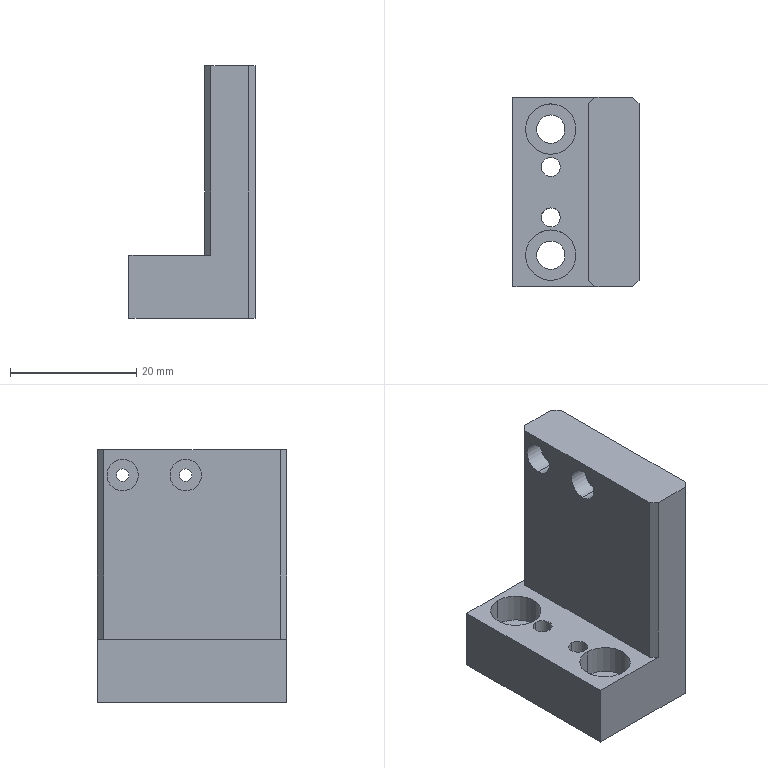Component | SolidWorks | JQ-2-0-007-3 | 1 solid | 36 faces | box 20 x 30 x 40 mm | volume 12205 mm3 | cylinder 20 | plane 16 | commonest cylinder face diameters 3 x4 2 x4 5 x4 8 x4 4.5 x4
STEP:
#1=COLOUR_RGB('',0.7922,0.8196,0.9333);
#2=FILL_AREA_STYLE_COLOUR('',#1);
#3=FILL_AREA_STYLE('',(#2));
#4=SURFACE_STYLE_FILL_AREA(#3);
#5=SURFACE_SIDE_STYLE('',(#4));
#6=SURFACE_STYLE_USAGE(.BOTH.,#5);
#7=PRESENTATION_STYLE_ASSIGNMENT((#6));
#8=CARTESIAN_POINT('',(-7.994,0.9385,4.611));
#9=VERTEX_POINT('',#8);
#10=CARTESIAN_POINT('',(-7.994,1.057,4.611));
#11=VERTEX_POINT('',#10);
#12=CARTESIAN_POINT('',(-7.994,0.9976,4.611));
#13=DIRECTION('',(0.,0.,1.));
#14=DIRECTION('',(0.,1.,0.));
#15=AXIS2_PLACEMENT_3D('',#12,#13,#14);
#16=CIRCLE('',#15,0.05906);
#17=EDGE_CURVE('',#9,#11,#16,.T.);
#18=ORIENTED_EDGE('',*,*,#17,.F.);
#19=CARTESIAN_POINT('',(-7.994,0.9385,5.005));
#20=VERTEX_POINT('',#19);
#21=CARTESIAN_POINT('',(-7.994,0.9385,4.611));
#22=DIRECTION('',(0.,0.,1.));
#23=VECTOR('',#22,39.37);
#24=LINE('',#21,#23);
#25=EDGE_CURVE('',#9,#20,#24,.T.);
#26=ORIENTED_EDGE('',*,*,#25,.T.);
#27=CARTESIAN_POINT('',(-7.994,1.057,5.005));
#28=VERTEX_POINT('',#27);
#29=CARTESIAN_POINT('',(-7.994,0.9976,5.005));
#30=DIRECTION('',(0.,0.,1.));
#31=DIRECTION('',(0.,1.,0.));
#32=AXIS2_PLACEMENT_3D('',#29,#30,#31);
#33=CIRCLE('',#32,0.05906);
#34=EDGE_CURVE('',#20,#28,#33,.T.);
#35=ORIENTED_EDGE('',*,*,#34,.T.);
#36=CARTESIAN_POINT('',(-7.994,1.057,4.611));
#37=DIRECTION('',(0.,0.,1.));
#38=VECTOR('',#37,39.37);
#39=LINE('',#36,#38);
#40=EDGE_CURVE('',#11,#28,#39,.T.);
#41=ORIENTED_EDGE('',*,*,#40,.F.);
#42=EDGE_LOOP('',(#18,#26,#35,#41));
#43=FACE_OUTER_BOUND('',#42,.T.);
#44=CARTESIAN_POINT('',(-7.994,0.9976,4.611));
#45=DIRECTION('',(0.,0.,1.));
#46=DIRECTION('',(0.,1.,0.));
#47=AXIS2_PLACEMENT_3D('',#44,#45,#46);
#48=CYLINDRICAL_SURFACE('',#47,0.05906);
#49=ADVANCED_FACE('',(#43),#48,.F.);
#50=CARTESIAN_POINT('',(-7.994,1.254,4.611));
#51=VERTEX_POINT('',#50);
#52=CARTESIAN_POINT('',(-7.994,1.372,4.611));
#53=VERTEX_POINT('',#52);
#54=CARTESIAN_POINT('',(-7.994,1.313,4.611));
#55=DIRECTION('',(0.,0.,1.));
#56=DIRECTION('',(0.,1.,0.));
#57=AXIS2_PLACEMENT_3D('',#54,#55,#56);
#58=CIRCLE('',#57,0.05906);
#59=EDGE_CURVE('',#51,#53,#58,.T.);
#60=ORIENTED_EDGE('',*,*,#59,.F.);
#61=CARTESIAN_POINT('',(-7.994,1.254,5.005));
#62=VERTEX_POINT('',#61);
#63=CARTESIAN_POINT('',(-7.994,1.254,4.611));
#64=DIRECTION('',(0.,0.,1.));
#65=VECTOR('',#64,39.37);
#66=LINE('',#63,#65);
#67=EDGE_CURVE('',#51,#62,#66,.T.);
#68=ORIENTED_EDGE('',*,*,#67,.T.);
#69=CARTESIAN_POINT('',(-7.994,1.372,5.005));
#70=VERTEX_POINT('',#69);
#71=CARTESIAN_POINT('',(-7.994,1.313,5.005));
#72=DIRECTION('',(0.,0.,1.));
#73=DIRECTION('',(0.,1.,0.));
#74=AXIS2_PLACEMENT_3D('',#71,#72,#73);
#75=CIRCLE('',#74,0.05906);
#76=EDGE_CURVE('',#62,#70,#75,.T.);
#77=ORIENTED_EDGE('',*,*,#76,.T.);
#78=CARTESIAN_POINT('',(-7.994,1.372,4.611));
#79=DIRECTION('',(0.,0.,1.));
#80=VECTOR('',#79,39.37);
#81=LINE('',#78,#80);
#82=EDGE_CURVE('',#53,#70,#81,.T.);
#83=ORIENTED_EDGE('',*,*,#82,.F.);
#84=EDGE_LOOP('',(#60,#68,#77,#83));
#85=FACE_OUTER_BOUND('',#84,.T.);
#86=CARTESIAN_POINT('',(-7.994,1.313,4.611));
#87=DIRECTION('',(0.,0.,1.));
#88=DIRECTION('',(0.,1.,0.));
#89=AXIS2_PLACEMENT_3D('',#86,#87,#88);
#90=CYLINDRICAL_SURFACE('',#89,0.05906);
#91=ADVANCED_FACE('',(#85),#90,.F.);
#92=CARTESIAN_POINT('',(-7.443,1.194,5.989));
#93=VERTEX_POINT('',#92);
#94=CARTESIAN_POINT('',(-7.443,1.194,6.068));
#95=VERTEX_POINT('',#94);
#96=CARTESIAN_POINT('',(-7.443,1.194,6.029));
#97=DIRECTION('',(-1.,-0.,0.));
#98=DIRECTION('',(0.,0.,1.));
#99=AXIS2_PLACEMENT_3D('',#96,#97,#98);
#100=CIRCLE('',#99,0.03937);
#101=EDGE_CURVE('',#93,#95,#100,.T.);
#102=ORIENTED_EDGE('',*,*,#101,.F.);
#103=CARTESIAN_POINT('',(-7.64,1.194,5.989));
#104=VERTEX_POINT('',#103);
#105=CARTESIAN_POINT('',(-7.443,1.194,5.989));
#106=DIRECTION('',(-1.,-0.,0.));
#107=VECTOR('',#106,39.37);
#108=LINE('',#105,#107);
#109=EDGE_CURVE('',#93,#104,#108,.T.);
#110=ORIENTED_EDGE('',*,*,#109,.T.);
#111=CARTESIAN_POINT('',(-7.64,1.194,6.068));
#112=VERTEX_POINT('',#111);
#113=CARTESIAN_POINT('',(-7.64,1.194,6.029));
#114=DIRECTION('',(-1.,-0.,0.));
#115=DIRECTION('',(0.,0.,1.));
#116=AXIS2_PLACEMENT_3D('',#113,#114,#115);
#117=CIRCLE('',#116,0.03937);
#118=EDGE_CURVE('',#104,#112,#117,.T.);
#119=ORIENTED_EDGE('',*,*,#118,.T.);
#120=CARTESIAN_POINT('',(-7.443,1.194,6.068));
#121=DIRECTION('',(-1.,-0.,0.));
#122=VECTOR('',#121,39.37);
#123=LINE('',#120,#122);
#124=EDGE_CURVE('',#95,#112,#123,.T.);
#125=ORIENTED_EDGE('',*,*,#124,.F.);
#126=EDGE_LOOP('',(#102,#110,#119,#125));
#127=FACE_OUTER_BOUND('',#126,.T.);
#128=CARTESIAN_POINT('',(-7.443,1.194,6.029));
#129=DIRECTION('',(-1.,-0.,0.));
#130=DIRECTION('',(0.,0.,1.));
#131=AXIS2_PLACEMENT_3D('',#128,#129,#130);
#132=CYLINDRICAL_SURFACE('',#131,0.03937);
#133=ADVANCED_FACE('',(#127),#132,.F.);
#134=CARTESIAN_POINT('',(-7.443,1.588,5.989));
#135=VERTEX_POINT('',#134);
#136=CARTESIAN_POINT('',(-7.443,1.588,6.068));
#137=VERTEX_POINT('',#136);
#138=CARTESIAN_POINT('',(-7.443,1.588,6.029));
#139=DIRECTION('',(-1.,-0.,0.));
#140=DIRECTION('',(0.,0.,1.));
#141=AXIS2_PLACEMENT_3D('',#138,#139,#140);
#142=CIRCLE('',#141,0.03937);
#143=EDGE_CURVE('',#135,#137,#142,.T.);
#144=ORIENTED_EDGE('',*,*,#143,.F.);
#145=CARTESIAN_POINT('',(-7.64,1.588,5.989));
#146=VERTEX_POINT('',#145);
#147=CARTESIAN_POINT('',(-7.443,1.588,5.989));
#148=DIRECTION('',(-1.,-0.,0.));
#149=VECTOR('',#148,39.37);
#150=LINE('',#147,#149);
#151=EDGE_CURVE('',#135,#146,#150,.T.);
#152=ORIENTED_EDGE('',*,*,#151,.T.);
#153=CARTESIAN_POINT('',(-7.64,1.588,6.068));
#154=VERTEX_POINT('',#153);
#155=CARTESIAN_POINT('',(-7.64,1.588,6.029));
#156=DIRECTION('',(-1.,-0.,0.));
#157=DIRECTION('',(0.,0.,1.));
#158=AXIS2_PLACEMENT_3D('',#155,#156,#157);
#159=CIRCLE('',#158,0.03937);
#160=EDGE_CURVE('',#146,#154,#159,.T.);
#161=ORIENTED_EDGE('',*,*,#160,.T.);
#162=CARTESIAN_POINT('',(-7.443,1.588,6.068));
#163=DIRECTION('',(-1.,-0.,0.));
#164=VECTOR('',#163,39.37);
#165=LINE('',#162,#164);
#166=EDGE_CURVE('',#137,#154,#165,.T.);
#167=ORIENTED_EDGE('',*,*,#166,.F.);
#168=EDGE_LOOP('',(#144,#152,#161,#167));
#169=FACE_OUTER_BOUND('',#168,.T.);
#170=CARTESIAN_POINT('',(-7.443,1.588,6.029));
#171=DIRECTION('',(-1.,-0.,0.));
#172=DIRECTION('',(0.,0.,1.));
#173=AXIS2_PLACEMENT_3D('',#170,#171,#172);
#174=CYLINDRICAL_SURFACE('',#173,0.03937);
#175=ADVANCED_FACE('',(#169),#174,.F.);
#176=CARTESIAN_POINT('',(-7.64,1.194,5.93));
#177=VERTEX_POINT('',#176);
#178=CARTESIAN_POINT('',(-7.64,1.194,6.127));
#179=VERTEX_POINT('',#178);
#180=CARTESIAN_POINT('',(-7.64,1.194,6.029));
#181=DIRECTION('',(-1.,-0.,0.));
#182=DIRECTION('',(0.,0.,1.));
#183=AXIS2_PLACEMENT_3D('',#180,#181,#182);
#184=CIRCLE('',#183,0.09843);
#185=EDGE_CURVE('',#177,#179,#184,.T.);
#186=ORIENTED_EDGE('',*,*,#185,.F.);
#187=CARTESIAN_POINT('',(-7.758,1.194,5.93));
#188=VERTEX_POINT('',#187);
#189=CARTESIAN_POINT('',(-7.64,1.194,5.93));
#190=DIRECTION('',(-1.,-0.,0.));
#191=VECTOR('',#190,39.37);
#192=LINE('',#189,#191);
#193=EDGE_CURVE('',#177,#188,#192,.T.);
#194=ORIENTED_EDGE('',*,*,#193,.T.);
#195=CARTESIAN_POINT('',(-7.758,1.194,6.127));
#196=VERTEX_POINT('',#195);
#197=CARTESIAN_POINT('',(-7.758,1.194,6.029));
#198=DIRECTION('',(-1.,-0.,0.));
#199=DIRECTION('',(0.,0.,1.));
#200=AXIS2_PLACEMENT_3D('',#197,#198,#199);
#201=CIRCLE('',#200,0.09843);
#202=EDGE_CURVE('',#188,#196,#201,.T.);
#203=ORIENTED_EDGE('',*,*,#202,.T.);
#204=CARTESIAN_POINT('',(-7.64,1.194,6.127));
#205=DIRECTION('',(-1.,-0.,0.));
#206=VECTOR('',#205,39.37);
#207=LINE('',#204,#206);
#208=EDGE_CURVE('',#179,#196,#207,.T.);
#209=ORIENTED_EDGE('',*,*,#208,.F.);
#210=EDGE_LOOP('',(#186,#194,#203,#209));
#211=FACE_OUTER_BOUND('',#210,.T.);
#212=CARTESIAN_POINT('',(-7.64,1.194,6.029));
#213=DIRECTION('',(-1.,-0.,0.));
#214=DIRECTION('',(0.,0.,1.));
#215=AXIS2_PLACEMENT_3D('',#212,#213,#214);
#216=CYLINDRICAL_SURFACE('',#215,0.09843);
#217=ADVANCED_FACE('',(#211),#216,.F.);
#218=CARTESIAN_POINT('',(-7.64,1.588,5.93));
#219=VERTEX_POINT('',#218);
#220=CARTESIAN_POINT('',(-7.64,1.588,6.127));
#221=VERTEX_POINT('',#220);
#222=CARTESIAN_POINT('',(-7.64,1.588,6.029));
#223=DIRECTION('',(-1.,-0.,0.));
#224=DIRECTION('',(0.,0.,1.));
#225=AXIS2_PLACEMENT_3D('',#222,#223,#224);
#226=CIRCLE('',#225,0.09843);
#227=EDGE_CURVE('',#219,#221,#226,.T.);
#228=ORIENTED_EDGE('',*,*,#227,.F.);
#229=CARTESIAN_POINT('',(-7.758,1.588,5.93));
#230=VERTEX_POINT('',#229);
#231=CARTESIAN_POINT('',(-7.64,1.588,5.93));
#232=DIRECTION('',(-1.,-0.,0.));
#233=VECTOR('',#232,39.37);
#234=LINE('',#231,#233);
#235=EDGE_CURVE('',#219,#230,#234,.T.);
#236=ORIENTED_EDGE('',*,*,#235,.T.);
#237=CARTESIAN_POINT('',(-7.758,1.588,6.127));
#238=VERTEX_POINT('',#237);
#239=CARTESIAN_POINT('',(-7.758,1.588,6.029));
#240=DIRECTION('',(-1.,-0.,0.));
#241=DIRECTION('',(0.,0.,1.));
#242=AXIS2_PLACEMENT_3D('',#239,#240,#241);
#243=CIRCLE('',#242,0.09843);
#244=EDGE_CURVE('',#230,#238,#243,.T.);
#245=ORIENTED_EDGE('',*,*,#244,.T.);
#246=CARTESIAN_POINT('',(-7.64,1.588,6.127));
#247=DIRECTION('',(-1.,-0.,0.));
#248=VECTOR('',#247,39.37);
#249=LINE('',#246,#248);
#250=EDGE_CURVE('',#221,#238,#249,.T.);
#251=ORIENTED_EDGE('',*,*,#250,.F.);
#252=EDGE_LOOP('',(#228,#236,#245,#251));
#253=FACE_OUTER_BOUND('',#252,.T.);
#254=CARTESIAN_POINT('',(-7.64,1.588,6.029));
#255=DIRECTION('',(-1.,-0.,0.));
#256=DIRECTION('',(0.,0.,1.));
#257=AXIS2_PLACEMENT_3D('',#254,#255,#256);
#258=CYLINDRICAL_SURFACE('',#257,0.09843);
#259=ADVANCED_FACE('',(#253),#258,.F.);
#260=CARTESIAN_POINT('',(-7.994,0.6039,4.824));
#261=VERTEX_POINT('',#260);
#262=CARTESIAN_POINT('',(-7.994,0.9189,4.824));
#263=VERTEX_POINT('',#262);
#264=CARTESIAN_POINT('',(-7.994,0.7614,4.824));
#265=DIRECTION('',(0.,0.,1.));
#266=DIRECTION('',(0.,1.,0.));
#267=AXIS2_PLACEMENT_3D('',#264,#265,#266);
#268=CIRCLE('',#267,0.1575);
#269=EDGE_CURVE('',#261,#263,#268,.T.);
#270=ORIENTED_EDGE('',*,*,#269,.F.);
#271=CARTESIAN_POINT('',(-7.994,0.6039,5.005));
#272=VERTEX_POINT('',#271);
#273=CARTESIAN_POINT('',(-7.994,0.6039,5.005));
#274=DIRECTION('',(0.,0.,1.));
#275=VECTOR('',#274,39.37);
#276=LINE('',#273,#275);
#277=EDGE_CURVE('',#261,#272,#276,.T.);
#278=ORIENTED_EDGE('',*,*,#277,.T.);
#279=CARTESIAN_POINT('',(-7.994,0.9189,5.005));
#280=VERTEX_POINT('',#279);
#281=CARTESIAN_POINT('',(-7.994,0.7614,5.005));
#282=DIRECTION('',(0.,0.,1.));
#283=DIRECTION('',(0.,1.,0.));
#284=AXIS2_PLACEMENT_3D('',#281,#282,#283);
#285=CIRCLE('',#284,0.1575);
#286=EDGE_CURVE('',#272,#280,#285,.T.);
#287=ORIENTED_EDGE('',*,*,#286,.T.);
#288=CARTESIAN_POINT('',(-7.994,0.9189,5.005));
#289=DIRECTION('',(0.,0.,1.));
#290=VECTOR('',#289,39.37);
#291=LINE('',#288,#290);
#292=EDGE_CURVE('',#263,#280,#291,.T.);
#293=ORIENTED_EDGE('',*,*,#292,.F.);
#294=EDGE_LOOP('',(#270,#278,#287,#293));
#295=FACE_OUTER_BOUND('',#294,.T.);
#296=CARTESIAN_POINT('',(-7.994,0.7614,5.005));
#297=DIRECTION('',(0.,0.,1.));
#298=DIRECTION('',(0.,1.,0.));
#299=AXIS2_PLACEMENT_3D('',#296,#297,#298);
#300=CYLINDRICAL_SURFACE('',#299,0.1575);
#301=ADVANCED_FACE('',(#295),#300,.F.);
#302=CARTESIAN_POINT('',(-7.994,0.6728,4.611));
#303=VERTEX_POINT('',#302);
#304=CARTESIAN_POINT('',(-7.994,0.85,4.611));
#305=VERTEX_POINT('',#304);
#306=CARTESIAN_POINT('',(-7.994,0.7614,4.611));
#307=DIRECTION('',(0.,0.,1.));
#308=DIRECTION('',(0.,1.,0.));
#309=AXIS2_PLACEMENT_3D('',#306,#307,#308);
#310=CIRCLE('',#309,0.08858);
#311=EDGE_CURVE('',#303,#305,#310,.T.);
#312=ORIENTED_EDGE('',*,*,#311,.F.);
#313=CARTESIAN_POINT('',(-7.994,0.6728,4.824));
#314=VERTEX_POINT('',#313);
#315=CARTESIAN_POINT('',(-7.994,0.6728,5.005));
#316=DIRECTION('',(0.,0.,1.));
#317=VECTOR('',#316,39.37);
#318=LINE('',#315,#317);
#319=EDGE_CURVE('',#303,#314,#318,.T.);
#320=ORIENTED_EDGE('',*,*,#319,.T.);
#321=CARTESIAN_POINT('',(-7.994,0.85,4.824));
#322=VERTEX_POINT('',#321);
#323=CARTESIAN_POINT('',(-7.994,0.7614,4.824));
#324=DIRECTION('',(0.,0.,1.));
#325=DIRECTION('',(0.,1.,0.));
#326=AXIS2_PLACEMENT_3D('',#323,#324,#325);
#327=CIRCLE('',#326,0.08858);
#328=EDGE_CURVE('',#314,#322,#327,.T.);
#329=ORIENTED_EDGE('',*,*,#328,.T.);
#330=CARTESIAN_POINT('',(-7.994,0.85,5.005));
#331=DIRECTION('',(0.,0.,1.));
#332=VECTOR('',#331,39.37);
#333=LINE('',#330,#332);
#334=EDGE_CURVE('',#305,#322,#333,.T.);
#335=ORIENTED_EDGE('',*,*,#334,.F.);
#336=EDGE_LOOP('',(#312,#320,#329,#335));
#337=FACE_OUTER_BOUND('',#336,.T.);
#338=CARTESIAN_POINT('',(-7.994,0.7614,5.005));
#339=DIRECTION('',(0.,0.,1.));
#340=DIRECTION('',(0.,1.,0.));
#341=AXIS2_PLACEMENT_3D('',#338,#339,#340);
#342=CYLINDRICAL_SURFACE('',#341,0.08858);
#343=ADVANCED_FACE('',(#337),#342,.F.);
#344=CARTESIAN_POINT('',(-7.994,1.391,4.824));
#345=VERTEX_POINT('',#344);
#346=CARTESIAN_POINT('',(-7.994,1.706,4.824));
#347=VERTEX_POINT('',#346);
#348=CARTESIAN_POINT('',(-7.994,1.549,4.824));
#349=DIRECTION('',(0.,0.,1.));
#350=DIRECTION('',(0.,1.,0.));
#351=AXIS2_PLACEMENT_3D('',#348,#349,#350);
#352=CIRCLE('',#351,0.1575);
#353=EDGE_CURVE('',#345,#347,#352,.T.);
#354=ORIENTED_EDGE('',*,*,#353,.F.);
#355=CARTESIAN_POINT('',(-7.994,1.391,5.005));
#356=VERTEX_POINT('',#355);
#357=CARTESIAN_POINT('',(-7.994,1.391,5.005));
#358=DIRECTION('',(0.,0.,1.));
#359=VECTOR('',#358,39.37);
#360=LINE('',#357,#359);
#361=EDGE_CURVE('',#345,#356,#360,.T.);
#362=ORIENTED_EDGE('',*,*,#361,.T.);
#363=CARTESIAN_POINT('',(-7.994,1.706,5.005));
#364=VERTEX_POINT('',#363);
#365=CARTESIAN_POINT('',(-7.994,1.549,5.005));
#366=DIRECTION('',(0.,0.,1.));
#367=DIRECTION('',(0.,1.,0.));
#368=AXIS2_PLACEMENT_3D('',#365,#366,#367);
#369=CIRCLE('',#368,0.1575);
#370=EDGE_CURVE('',#356,#364,#369,.T.);
#371=ORIENTED_EDGE('',*,*,#370,.T.);
#372=CARTESIAN_POINT('',(-7.994,1.706,5.005));
#373=DIRECTION('',(0.,0.,1.));
#374=VECTOR('',#373,39.37);
#375=LINE('',#372,#374);
#376=EDGE_CURVE('',#347,#364,#375,.T.);
#377=ORIENTED_EDGE('',*,*,#376,.F.);
#378=EDGE_LOOP('',(#354,#362,#371,#377));
#379=FACE_OUTER_BOUND('',#378,.T.);
#380=CARTESIAN_POINT('',(-7.994,1.549,5.005));
#381=DIRECTION('',(0.,0.,1.));
#382=DIRECTION('',(0.,1.,0.));
#383=AXIS2_PLACEMENT_3D('',#380,#381,#382);
#384=CYLINDRICAL_SURFACE('',#383,0.1575);
#385=ADVANCED_FACE('',(#379),#384,.F.);
#386=CARTESIAN_POINT('',(-7.994,1.46,4.611));
#387=VERTEX_POINT('',#386);
#388=CARTESIAN_POINT('',(-7.994,1.637,4.611));
#389=VERTEX_POINT('',#388);
#390=CARTESIAN_POINT('',(-7.994,1.549,4.611));
#391=DIRECTION('',(0.,0.,1.));
#392=DIRECTION('',(0.,1.,0.));
#393=AXIS2_PLACEMENT_3D('',#390,#391,#392);
#394=CIRCLE('',#393,0.08858);
#395=EDGE_CURVE('',#387,#389,#394,.T.);
#396=ORIENTED_EDGE('',*,*,#395,.F.);
#397=CARTESIAN_POINT('',(-7.994,1.46,4.824));
#398=VERTEX_POINT('',#397);
#399=CARTESIAN_POINT('',(-7.994,1.46,5.005));
#400=DIRECTION('',(0.,0.,1.));
#401=VECTOR('',#400,39.37);
#402=LINE('',#399,#401);
#403=EDGE_CURVE('',#387,#398,#402,.T.);
#404=ORIENTED_EDGE('',*,*,#403,.T.);
#405=CARTESIAN_POINT('',(-7.994,1.637,4.824));
#406=VERTEX_POINT('',#405);
#407=CARTESIAN_POINT('',(-7.994,1.549,4.824));
#408=DIRECTION('',(0.,0.,1.));
#409=DIRECTION('',(0.,1.,0.));
#410=AXIS2_PLACEMENT_3D('',#407,#408,#409);
#411=CIRCLE('',#410,0.08858);
#412=EDGE_CURVE('',#398,#406,#411,.T.);
#413=ORIENTED_EDGE('',*,*,#412,.T.);
#414=CARTESIAN_POINT('',(-7.994,1.637,5.005));
#415=DIRECTION('',(0.,0.,1.));
#416=VECTOR('',#415,39.37);
#417=LINE('',#414,#416);
#418=EDGE_CURVE('',#389,#406,#417,.T.);
#419=ORIENTED_EDGE('',*,*,#418,.F.);
#420=EDGE_LOOP('',(#396,#404,#413,#419));
#421=FACE_OUTER_BOUND('',#420,.T.);
#422=CARTESIAN_POINT('',(-7.994,1.549,5.005));
#423=DIRECTION('',(0.,0.,1.));
#424=DIRECTION('',(0.,1.,0.));
#425=AXIS2_PLACEMENT_3D('',#422,#423,#424);
#426=CYLINDRICAL_SURFACE('',#425,0.08858);
#427=ADVANCED_FACE('',(#421),#426,.F.);
#428=CARTESIAN_POINT('',(-7.994,0.9976,4.611));
#429=DIRECTION('',(0.,0.,1.));
#430=DIRECTION('',(0.,1.,0.));
#431=AXIS2_PLACEMENT_3D('',#428,#429,#430);
#432=CIRCLE('',#431,0.05906);
#433=EDGE_CURVE('',#11,#9,#432,.T.);
#434=ORIENTED_EDGE('',*,*,#433,.T.);
#435=ORIENTED_EDGE('',*,*,#17,.T.);
#436=EDGE_LOOP('',(#434,#435));
#437=FACE_BOUND('',#436,.T.);
#438=CARTESIAN_POINT('',(-7.994,1.313,4.611));
#439=DIRECTION('',(0.,0.,1.));
#440=DIRECTION('',(0.,1.,0.));
#441=AXIS2_PLACEMENT_3D('',#438,#439,#440);
#442=CIRCLE('',#441,0.05906);
#443=EDGE_CURVE('',#53,#51,#442,.T.);
#444=ORIENTED_EDGE('',*,*,#443,.T.);
#445=ORIENTED_EDGE('',*,*,#59,.T.);
#446=EDGE_LOOP('',(#444,#445));
#447=FACE_BOUND('',#446,.T.);
#448=CARTESIAN_POINT('',(-7.994,0.7614,4.611));
#449=DIRECTION('',(0.,0.,1.));
#450=DIRECTION('',(0.,1.,0.));
#451=AXIS2_PLACEMENT_3D('',#448,#449,#450);
#452=CIRCLE('',#451,0.08858);
#453=EDGE_CURVE('',#305,#303,#452,.T.);
#454=ORIENTED_EDGE('',*,*,#453,.T.);
#455=ORIENTED_EDGE('',*,*,#311,.T.);
#456=EDGE_LOOP('',(#454,#455));
#457=FACE_BOUND('',#456,.T.);
#458=CARTESIAN_POINT('',(-7.994,1.549,4.611));
#459=DIRECTION('',(0.,0.,1.));
#460=DIRECTION('',(0.,1.,0.));
#461=AXIS2_PLACEMENT_3D('',#458,#459,#460);
#462=CIRCLE('',#461,0.08858);
#463=EDGE_CURVE('',#389,#387,#462,.T.);
#464=ORIENTED_EDGE('',*,*,#463,.T.);
#465=ORIENTED_EDGE('',*,*,#395,.T.);
#466=EDGE_LOOP('',(#464,#465));
#467=FACE_BOUND('',#466,.T.);
#468=CARTESIAN_POINT('',(-7.443,1.706,4.611));
#469=VERTEX_POINT('',#468);
#470=CARTESIAN_POINT('',(-7.443,0.6039,4.611));
#471=VERTEX_POINT('',#470);
#472=CARTESIAN_POINT('',(-7.443,1.746,4.611));
#473=DIRECTION('',(0.,-1.,0.));
#474=VECTOR('',#473,39.37);
#475=LINE('',#472,#474);
#476=EDGE_CURVE('',#469,#471,#475,.T.);
#477=ORIENTED_EDGE('',*,*,#476,.T.);
#478=CARTESIAN_POINT('',(-7.483,0.5645,4.611));
#479=VERTEX_POINT('',#478);
#480=CARTESIAN_POINT('',(-7.443,0.6039,4.611));
#481=DIRECTION('',(-0.7071,-0.7071,0.));
#482=VECTOR('',#481,39.37);
#483=LINE('',#480,#482);
#484=EDGE_CURVE('',#471,#479,#483,.T.);
#485=ORIENTED_EDGE('',*,*,#484,.T.);
#486=CARTESIAN_POINT('',(-8.231,0.5645,4.611));
#487=VERTEX_POINT('',#486);
#488=CARTESIAN_POINT('',(-8.231,0.5645,4.611));
#489=DIRECTION('',(-1.,-0.,0.));
#490=VECTOR('',#489,39.37);
#491=LINE('',#488,#490);
#492=EDGE_CURVE('',#479,#487,#491,.T.);
#493=ORIENTED_EDGE('',*,*,#492,.T.);
#494=CARTESIAN_POINT('',(-8.231,1.746,4.611));
#495=VERTEX_POINT('',#494);
#496=CARTESIAN_POINT('',(-8.231,1.746,4.611));
#497=DIRECTION('',(0.,-1.,0.));
#498=VECTOR('',#497,39.37);
#499=LINE('',#496,#498);
#500=EDGE_CURVE('',#495,#487,#499,.T.);
#501=ORIENTED_EDGE('',*,*,#500,.F.);
#502=CARTESIAN_POINT('',(-7.483,1.746,4.611));
#503=VERTEX_POINT('',#502);
#504=CARTESIAN_POINT('',(-8.231,1.746,4.611));
#505=DIRECTION('',(-1.,-0.,0.));
#506=VECTOR('',#505,39.37);
#507=LINE('',#504,#506);
#508=EDGE_CURVE('',#503,#495,#507,.T.);
#509=ORIENTED_EDGE('',*,*,#508,.F.);
#510=CARTESIAN_POINT('',(-7.483,1.746,4.611));
#511=DIRECTION('',(0.7071,-0.7071,0.));
#512=VECTOR('',#511,39.37);
#513=LINE('',#510,#512);
#514=EDGE_CURVE('',#503,#469,#513,.T.);
#515=ORIENTED_EDGE('',*,*,#514,.T.);
#516=EDGE_LOOP('',(#477,#485,#493,#501,#509,#515));
#517=FACE_OUTER_BOUND('',#516,.T.);
#518=CARTESIAN_POINT('',(-8.231,1.746,4.611));
#519=DIRECTION('',(0.,0.,1.));
#520=DIRECTION('',(1.,0.,-0.));
#521=AXIS2_PLACEMENT_3D('',#518,#519,#520);
#522=PLANE('',#521);
#523=ADVANCED_FACE('',(#437,#447,#457,#467,#517),#522,.F.);
#524=CARTESIAN_POINT('',(-8.231,0.5645,5.005));
#525=VERTEX_POINT('',#524);
#526=CARTESIAN_POINT('',(-8.231,0.5645,5.005));
#527=DIRECTION('',(0.,0.,1.));
#528=VECTOR('',#527,39.37);
#529=LINE('',#526,#528);
#530=EDGE_CURVE('',#487,#525,#529,.T.);
#531=ORIENTED_EDGE('',*,*,#530,.T.);
#532=CARTESIAN_POINT('',(-8.231,1.746,5.005));
#533=VERTEX_POINT('',#532);
#534=CARTESIAN_POINT('',(-8.231,1.746,5.005));
#535=DIRECTION('',(0.,-1.,0.));
#536=VECTOR('',#535,39.37);
#537=LINE('',#534,#536);
#538=EDGE_CURVE('',#533,#525,#537,.T.);
#539=ORIENTED_EDGE('',*,*,#538,.F.);
#540=CARTESIAN_POINT('',(-8.231,1.746,5.005));
#541=DIRECTION('',(0.,0.,1.));
#542=VECTOR('',#541,39.37);
#543=LINE('',#540,#542);
#544=EDGE_CURVE('',#495,#533,#543,.T.);
#545=ORIENTED_EDGE('',*,*,#544,.F.);
#546=ORIENTED_EDGE('',*,*,#500,.T.);
#547=EDGE_LOOP('',(#531,#539,#545,#546));
#548=FACE_OUTER_BOUND('',#547,.T.);
#549=CARTESIAN_POINT('',(-8.231,1.746,5.005));
#550=DIRECTION('',(1.,0.,-0.));
#551=DIRECTION('',(-0.,1.,-0.));
#552=AXIS2_PLACEMENT_3D('',#549,#550,#551);
#553=PLANE('',#552);
#554=ADVANCED_FACE('',(#548),#553,.F.);
#555=CARTESIAN_POINT('',(-7.994,0.9976,5.005));
#556=DIRECTION('',(0.,0.,1.));
#557=DIRECTION('',(0.,1.,0.));
#558=AXIS2_PLACEMENT_3D('',#555,#556,#557);
#559=CIRCLE('',#558,0.05906);
#560=EDGE_CURVE('',#28,#20,#559,.T.);
#561=ORIENTED_EDGE('',*,*,#560,.F.);
#562=ORIENTED_EDGE('',*,*,#34,.F.);
#563=EDGE_LOOP('',(#561,#562));
#564=FACE_BOUND('',#563,.T.);
#565=CARTESIAN_POINT('',(-7.994,1.313,5.005));
#566=DIRECTION('',(0.,0.,1.));
#567=DIRECTION('',(0.,1.,0.));
#568=AXIS2_PLACEMENT_3D('',#565,#566,#567);
#569=CIRCLE('',#568,0.05906);
#570=EDGE_CURVE('',#70,#62,#569,.T.);
#571=ORIENTED_EDGE('',*,*,#570,.F.);
#572=ORIENTED_EDGE('',*,*,#76,.F.);
#573=EDGE_LOOP('',(#571,#572));
#574=FACE_BOUND('',#573,.T.);
#575=CARTESIAN_POINT('',(-7.994,0.7614,5.005));
#576=DIRECTION('',(0.,0.,1.));
#577=DIRECTION('',(0.,1.,0.));
#578=AXIS2_PLACEMENT_3D('',#575,#576,#577);
#579=CIRCLE('',#578,0.1575);
#580=EDGE_CURVE('',#280,#272,#579,.T.);
#581=ORIENTED_EDGE('',*,*,#580,.F.);
#582=ORIENTED_EDGE('',*,*,#286,.F.);
#583=EDGE_LOOP('',(#581,#582));
#584=FACE_BOUND('',#583,.T.);
#585=CARTESIAN_POINT('',(-7.994,1.549,5.005));
#586=DIRECTION('',(0.,0.,1.));
#587=DIRECTION('',(0.,1.,0.));
#588=AXIS2_PLACEMENT_3D('',#585,#586,#587);
#589=CIRCLE('',#588,0.1575);
#590=EDGE_CURVE('',#364,#356,#589,.T.);
#591=ORIENTED_EDGE('',*,*,#590,.F.);
#592=ORIENTED_EDGE('',*,*,#370,.F.);
#593=EDGE_LOOP('',(#591,#592));
#594=FACE_BOUND('',#593,.T.);
#595=CARTESIAN_POINT('',(-7.719,0.5645,5.005));
#596=VERTEX_POINT('',#595);
#597=CARTESIAN_POINT('',(-7.758,0.5645,5.005));
#598=DIRECTION('',(1.,0.,-0.));
#599=VECTOR('',#598,39.37);
#600=LINE('',#597,#599);
#601=EDGE_CURVE('',#525,#596,#600,.T.);
#602=ORIENTED_EDGE('',*,*,#601,.T.);
#603=CARTESIAN_POINT('',(-7.758,0.6039,5.005));
#604=VERTEX_POINT('',#603);
#605=CARTESIAN_POINT('',(-8.329,1.175,5.005));
#606=DIRECTION('',(-0.7071,0.7071,-0.));
#607=VECTOR('',#606,39.37);
#608=LINE('',#605,#607);
#609=EDGE_CURVE('',#596,#604,#608,.T.);
#610=ORIENTED_EDGE('',*,*,#609,.T.);
#611=CARTESIAN_POINT('',(-7.758,1.706,5.005));
#612=VERTEX_POINT('',#611);
#613=CARTESIAN_POINT('',(-7.758,1.746,5.005));
#614=DIRECTION('',(0.,-1.,0.));
#615=VECTOR('',#614,39.37);
#616=LINE('',#613,#615);
#617=EDGE_CURVE('',#612,#604,#616,.T.);
#618=ORIENTED_EDGE('',*,*,#617,.F.);
#619=CARTESIAN_POINT('',(-7.719,1.746,5.005));
#620=VERTEX_POINT('',#619);
#621=CARTESIAN_POINT('',(-7.739,1.726,5.005));
#622=DIRECTION('',(0.7071,0.7071,-0.));
#623=VECTOR('',#622,39.37);
#624=LINE('',#621,#623);
#625=EDGE_CURVE('',#612,#620,#624,.T.);
#626=ORIENTED_EDGE('',*,*,#625,.T.);
#627=CARTESIAN_POINT('',(-7.758,1.746,5.005));
#628=DIRECTION('',(1.,0.,-0.));
#629=VECTOR('',#628,39.37);
#630=LINE('',#627,#629);
#631=EDGE_CURVE('',#533,#620,#630,.T.);
#632=ORIENTED_EDGE('',*,*,#631,.F.);
#633=ORIENTED_EDGE('',*,*,#538,.T.);
#634=EDGE_LOOP('',(#602,#610,#618,#626,#632,#633));
#635=FACE_OUTER_BOUND('',#634,.T.);
#636=CARTESIAN_POINT('',(-7.758,1.746,5.005));
#637=DIRECTION('',(-0.,-0.,-1.));
#638=DIRECTION('',(0.,-1.,0.));
#639=AXIS2_PLACEMENT_3D('',#636,#637,#638);
#640=PLANE('',#639);
#641=ADVANCED_FACE('',(#564,#574,#584,#594,#635),#640,.F.);
#642=CARTESIAN_POINT('',(-7.758,1.194,6.029));
#643=DIRECTION('',(-1.,-0.,0.));
#644=DIRECTION('',(0.,0.,1.));
#645=AXIS2_PLACEMENT_3D('',#642,#643,#644);
#646=CIRCLE('',#645,0.09843);
#647=EDGE_CURVE('',#196,#188,#646,.T.);
#648=ORIENTED_EDGE('',*,*,#647,.F.);
#649=ORIENTED_EDGE('',*,*,#202,.F.);
#650=EDGE_LOOP('',(#648,#649));
#651=FACE_BOUND('',#650,.T.);
#652=CARTESIAN_POINT('',(-7.758,1.588,6.029));
#653=DIRECTION('',(-1.,-0.,0.));
#654=DIRECTION('',(0.,0.,1.));
#655=AXIS2_PLACEMENT_3D('',#652,#653,#654);
#656=CIRCLE('',#655,0.09843);
#657=EDGE_CURVE('',#238,#230,#656,.T.);
#658=ORIENTED_EDGE('',*,*,#657,.F.);
#659=ORIENTED_EDGE('',*,*,#244,.F.);
#660=EDGE_LOOP('',(#658,#659));
#661=FACE_BOUND('',#660,.T.);
#662=ORIENTED_EDGE('',*,*,#617,.T.);
#663=CARTESIAN_POINT('',(-7.758,0.6039,6.186));
#664=VERTEX_POINT('',#663);
#665=CARTESIAN_POINT('',(-7.758,0.6039,6.186));
#666=DIRECTION('',(0.,0.,1.));
#667=VECTOR('',#666,39.37);
#668=LINE('',#665,#667);
#669=EDGE_CURVE('',#604,#664,#668,.T.);
#670=ORIENTED_EDGE('',*,*,#669,.T.);
#671=CARTESIAN_POINT('',(-7.758,1.706,6.186));
#672=VERTEX_POINT('',#671);
#673=CARTESIAN_POINT('',(-7.758,1.746,6.186));
#674=DIRECTION('',(0.,-1.,0.));
#675=VECTOR('',#674,39.37);
#676=LINE('',#673,#675);
#677=EDGE_CURVE('',#672,#664,#676,.T.);
#678=ORIENTED_EDGE('',*,*,#677,.F.);
#679=CARTESIAN_POINT('',(-7.758,1.706,6.186));
#680=DIRECTION('',(-0.,-0.,-1.));
#681=VECTOR('',#680,39.37);
#682=LINE('',#679,#681);
#683=EDGE_CURVE('',#672,#612,#682,.T.);
#684=ORIENTED_EDGE('',*,*,#683,.T.);
#685=EDGE_LOOP('',(#662,#670,#678,#684));
#686=FACE_OUTER_BOUND('',#685,.T.);
#687=CARTESIAN_POINT('',(-7.758,1.746,6.186));
#688=DIRECTION('',(1.,0.,-0.));
#689=DIRECTION('',(-0.,-0.,-1.));
#690=AXIS2_PLACEMENT_3D('',#687,#688,#689);
#691=PLANE('',#690);
#692=ADVANCED_FACE('',(#651,#661,#686),#691,.F.);
#693=CARTESIAN_POINT('',(-7.719,0.5645,6.186));
#694=VERTEX_POINT('',#693);
#695=CARTESIAN_POINT('',(-7.483,0.5645,6.186));
#696=VERTEX_POINT('',#695);
#697=CARTESIAN_POINT('',(-7.443,0.5645,6.186));
#698=DIRECTION('',(1.,0.,-0.));
#699=VECTOR('',#698,39.37);
#700=LINE('',#697,#699);
#701=EDGE_CURVE('',#694,#696,#700,.T.);
#702=ORIENTED_EDGE('',*,*,#701,.T.);
#703=CARTESIAN_POINT('',(-7.443,0.6039,6.186));
#704=VERTEX_POINT('',#703);
#705=CARTESIAN_POINT('',(-7.443,0.6039,6.186));
#706=DIRECTION('',(0.7071,0.7071,-0.));
#707=VECTOR('',#706,39.37);
#708=LINE('',#705,#707);
#709=EDGE_CURVE('',#696,#704,#708,.T.);
#710=ORIENTED_EDGE('',*,*,#709,.T.);
#711=CARTESIAN_POINT('',(-7.443,1.706,6.186));
#712=VERTEX_POINT('',#711);
#713=CARTESIAN_POINT('',(-7.443,1.746,6.186));
#714=DIRECTION('',(0.,-1.,0.));
#715=VECTOR('',#714,39.37);
#716=LINE('',#713,#715);
#717=EDGE_CURVE('',#712,#704,#716,.T.);
#718=ORIENTED_EDGE('',*,*,#717,.F.);
#719=CARTESIAN_POINT('',(-7.483,1.746,6.186));
#720=VERTEX_POINT('',#719);
#721=CARTESIAN_POINT('',(-7.483,1.746,6.186));
#722=DIRECTION('',(-0.7071,0.7071,-0.));
#723=VECTOR('',#722,39.37);
#724=LINE('',#721,#723);
#725=EDGE_CURVE('',#712,#720,#724,.T.);
#726=ORIENTED_EDGE('',*,*,#725,.T.);
#727=CARTESIAN_POINT('',(-7.719,1.746,6.186));
#728=VERTEX_POINT('',#727);
#729=CARTESIAN_POINT('',(-7.443,1.746,6.186));
#730=DIRECTION('',(1.,0.,-0.));
#731=VECTOR('',#730,39.37);
#732=LINE('',#729,#731);
#733=EDGE_CURVE('',#728,#720,#732,.T.);
#734=ORIENTED_EDGE('',*,*,#733,.F.);
#735=CARTESIAN_POINT('',(-7.719,1.746,6.186));
#736=DIRECTION('',(-0.7071,-0.7071,0.));
#737=VECTOR('',#736,39.37);
#738=LINE('',#735,#737);
#739=EDGE_CURVE('',#728,#672,#738,.T.);
#740=ORIENTED_EDGE('',*,*,#739,.T.);
#741=ORIENTED_EDGE('',*,*,#677,.T.);
#742=CARTESIAN_POINT('',(-7.758,0.6039,6.186));
#743=DIRECTION('',(0.7071,-0.7071,0.));
#744=VECTOR('',#743,39.37);
#745=LINE('',#742,#744);
#746=EDGE_CURVE('',#664,#694,#745,.T.);
#747=ORIENTED_EDGE('',*,*,#746,.T.);
#748=EDGE_LOOP('',(#702,#710,#718,#726,#734,#740,#741,#747));
#749=FACE_OUTER_BOUND('',#748,.T.);
#750=CARTESIAN_POINT('',(-7.443,1.746,6.186));
#751=DIRECTION('',(-0.,-0.,-1.));
#752=DIRECTION('',(0.,-1.,0.));
#753=AXIS2_PLACEMENT_3D('',#750,#751,#752);
#754=PLANE('',#753);
#755=ADVANCED_FACE('',(#749),#754,.F.);
#756=CARTESIAN_POINT('',(-7.443,1.194,6.029));
#757=DIRECTION('',(-1.,-0.,0.));
#758=DIRECTION('',(0.,0.,1.));
#759=AXIS2_PLACEMENT_3D('',#756,#757,#758);
#760=CIRCLE('',#759,0.03937);
#761=EDGE_CURVE('',#95,#93,#760,.T.);
#762=ORIENTED_EDGE('',*,*,#761,.T.);
#763=ORIENTED_EDGE('',*,*,#101,.T.);
#764=EDGE_LOOP('',(#762,#763));
#765=FACE_BOUND('',#764,.T.);
#766=CARTESIAN_POINT('',(-7.443,1.588,6.029));
#767=DIRECTION('',(-1.,-0.,0.));
#768=DIRECTION('',(0.,0.,1.));
#769=AXIS2_PLACEMENT_3D('',#766,#767,#768);
#770=CIRCLE('',#769,0.03937);
#771=EDGE_CURVE('',#137,#135,#770,.T.);
#772=ORIENTED_EDGE('',*,*,#771,.T.);
#773=ORIENTED_EDGE('',*,*,#143,.T.);
#774=EDGE_LOOP('',(#772,#773));
#775=FACE_BOUND('',#774,.T.);
#776=ORIENTED_EDGE('',*,*,#717,.T.);
#777=CARTESIAN_POINT('',(-7.443,0.6039,4.611));
#778=DIRECTION('',(-0.,-0.,-1.));
#779=VECTOR('',#778,39.37);
#780=LINE('',#777,#779);
#781=EDGE_CURVE('',#704,#471,#780,.T.);
#782=ORIENTED_EDGE('',*,*,#781,.T.);
#783=ORIENTED_EDGE('',*,*,#476,.F.);
#784=CARTESIAN_POINT('',(-7.443,1.706,4.611));
#785=DIRECTION('',(0.,0.,1.));
#786=VECTOR('',#785,39.37);
#787=LINE('',#784,#786);
#788=EDGE_CURVE('',#469,#712,#787,.T.);
#789=ORIENTED_EDGE('',*,*,#788,.T.);
#790=EDGE_LOOP('',(#776,#782,#783,#789));
#791=FACE_OUTER_BOUND('',#790,.T.);
#792=CARTESIAN_POINT('',(-7.443,1.746,4.611));
#793=DIRECTION('',(-1.,-0.,0.));
#794=DIRECTION('',(0.,-1.,0.));
#795=AXIS2_PLACEMENT_3D('',#792,#793,#794);
#796=PLANE('',#795);
#797=ADVANCED_FACE('',(#765,#775,#791),#796,.F.);
#798=ORIENTED_EDGE('',*,*,#733,.T.);
#799=CARTESIAN_POINT('',(-7.483,1.746,4.611));
#800=DIRECTION('',(-0.,-0.,-1.));
#801=VECTOR('',#800,39.37);
#802=LINE('',#799,#801);
#803=EDGE_CURVE('',#720,#503,#802,.T.);
#804=ORIENTED_EDGE('',*,*,#803,.T.);
#805=ORIENTED_EDGE('',*,*,#508,.T.);
#806=ORIENTED_EDGE('',*,*,#544,.T.);
#807=ORIENTED_EDGE('',*,*,#631,.T.);
#808=CARTESIAN_POINT('',(-7.719,1.746,4.611));
#809=DIRECTION('',(0.,0.,1.));
#810=VECTOR('',#809,39.37);
#811=LINE('',#808,#810);
#812=EDGE_CURVE('',#620,#728,#811,.T.);
#813=ORIENTED_EDGE('',*,*,#812,.T.);
#814=EDGE_LOOP('',(#798,#804,#805,#806,#807,#813));
#815=FACE_OUTER_BOUND('',#814,.T.);
#816=CARTESIAN_POINT('',(-7.443,1.746,4.611));
#817=DIRECTION('',(0.,-1.,0.));
#818=DIRECTION('',(1.,0.,-0.));
#819=AXIS2_PLACEMENT_3D('',#816,#817,#818);
#820=PLANE('',#819);
#821=ADVANCED_FACE('',(#815),#820,.F.);
#822=ORIENTED_EDGE('',*,*,#492,.F.);
#823=CARTESIAN_POINT('',(-7.483,0.5645,6.186));
#824=DIRECTION('',(0.,0.,1.));
#825=VECTOR('',#824,39.37);
#826=LINE('',#823,#825);
#827=EDGE_CURVE('',#479,#696,#826,.T.);
#828=ORIENTED_EDGE('',*,*,#827,.T.);
#829=ORIENTED_EDGE('',*,*,#701,.F.);
#830=CARTESIAN_POINT('',(-7.719,0.5645,5.005));
#831=DIRECTION('',(-0.,-0.,-1.));
#832=VECTOR('',#831,39.37);
#833=LINE('',#830,#832);
#834=EDGE_CURVE('',#694,#596,#833,.T.);
#835=ORIENTED_EDGE('',*,*,#834,.T.);
#836=ORIENTED_EDGE('',*,*,#601,.F.);
#837=ORIENTED_EDGE('',*,*,#530,.F.);
#838=EDGE_LOOP('',(#822,#828,#829,#835,#836,#837));
#839=FACE_OUTER_BOUND('',#838,.T.);
#840=CARTESIAN_POINT('',(-7.443,0.5645,4.611));
#841=DIRECTION('',(0.,-1.,0.));
#842=DIRECTION('',(1.,0.,-0.));
#843=AXIS2_PLACEMENT_3D('',#840,#841,#842);
#844=PLANE('',#843);
#845=ADVANCED_FACE('',(#839),#844,.T.);
#846=ORIENTED_EDGE('',*,*,#403,.F.);
#847=ORIENTED_EDGE('',*,*,#463,.F.);
#848=ORIENTED_EDGE('',*,*,#418,.T.);
#849=CARTESIAN_POINT('',(-7.994,1.549,4.824));
#850=DIRECTION('',(0.,0.,1.));
#851=DIRECTION('',(0.,1.,0.));
#852=AXIS2_PLACEMENT_3D('',#849,#850,#851);
#853=CIRCLE('',#852,0.08858);
#854=EDGE_CURVE('',#406,#398,#853,.T.);
#855=ORIENTED_EDGE('',*,*,#854,.T.);
#856=EDGE_LOOP('',(#846,#847,#848,#855));
#857=FACE_OUTER_BOUND('',#856,.T.);
#858=CARTESIAN_POINT('',(-7.994,1.549,5.005));
#859=DIRECTION('',(0.,0.,1.));
#860=DIRECTION('',(0.,1.,0.));
#861=AXIS2_PLACEMENT_3D('',#858,#859,#860);
#862=CYLINDRICAL_SURFACE('',#861,0.08858);
#863=ADVANCED_FACE('',(#857),#862,.F.);
#864=ORIENTED_EDGE('',*,*,#854,.F.);
#865=ORIENTED_EDGE('',*,*,#412,.F.);
#866=EDGE_LOOP('',(#864,#865));
#867=FACE_BOUND('',#866,.T.);
#868=CARTESIAN_POINT('',(-7.994,1.549,4.824));
#869=DIRECTION('',(0.,0.,1.));
#870=DIRECTION('',(0.,1.,0.));
#871=AXIS2_PLACEMENT_3D('',#868,#869,#870);
#872=CIRCLE('',#871,0.1575);
#873=EDGE_CURVE('',#347,#345,#872,.T.);
#874=ORIENTED_EDGE('',*,*,#873,.T.);
#875=ORIENTED_EDGE('',*,*,#353,.T.);
#876=EDGE_LOOP('',(#874,#875));
#877=FACE_OUTER_BOUND('',#876,.T.);
#878=CARTESIAN_POINT('',(-8.083,1.549,4.824));
#879=DIRECTION('',(-0.,-0.,-1.));
#880=DIRECTION('',(0.,-1.,0.));
#881=AXIS2_PLACEMENT_3D('',#878,#879,#880);
#882=PLANE('',#881);
#883=ADVANCED_FACE('',(#867,#877),#882,.F.);
#884=ORIENTED_EDGE('',*,*,#361,.F.);
#885=ORIENTED_EDGE('',*,*,#873,.F.);
#886=ORIENTED_EDGE('',*,*,#376,.T.);
#887=ORIENTED_EDGE('',*,*,#590,.T.);
#888=EDGE_LOOP('',(#884,#885,#886,#887));
#889=FACE_OUTER_BOUND('',#888,.T.);
#890=CARTESIAN_POINT('',(-7.994,1.549,5.005));
#891=DIRECTION('',(0.,0.,1.));
#892=DIRECTION('',(0.,1.,0.));
#893=AXIS2_PLACEMENT_3D('',#890,#891,#892);
#894=CYLINDRICAL_SURFACE('',#893,0.1575);
#895=ADVANCED_FACE('',(#889),#894,.F.);
#896=ORIENTED_EDGE('',*,*,#319,.F.);
#897=ORIENTED_EDGE('',*,*,#453,.F.);
#898=ORIENTED_EDGE('',*,*,#334,.T.);
#899=CARTESIAN_POINT('',(-7.994,0.7614,4.824));
#900=DIRECTION('',(0.,0.,1.));
#901=DIRECTION('',(0.,1.,0.));
#902=AXIS2_PLACEMENT_3D('',#899,#900,#901);
#903=CIRCLE('',#902,0.08858);
#904=EDGE_CURVE('',#322,#314,#903,.T.);
#905=ORIENTED_EDGE('',*,*,#904,.T.);
#906=EDGE_LOOP('',(#896,#897,#898,#905));
#907=FACE_OUTER_BOUND('',#906,.T.);
#908=CARTESIAN_POINT('',(-7.994,0.7614,5.005));
#909=DIRECTION('',(0.,0.,1.));
#910=DIRECTION('',(0.,1.,0.));
#911=AXIS2_PLACEMENT_3D('',#908,#909,#910);
#912=CYLINDRICAL_SURFACE('',#911,0.08858);
#913=ADVANCED_FACE('',(#907),#912,.F.);
#914=ORIENTED_EDGE('',*,*,#904,.F.);
#915=ORIENTED_EDGE('',*,*,#328,.F.);
#916=EDGE_LOOP('',(#914,#915));
#917=FACE_BOUND('',#916,.T.);
#918=CARTESIAN_POINT('',(-7.994,0.7614,4.824));
#919=DIRECTION('',(0.,0.,1.));
#920=DIRECTION('',(0.,1.,0.));
#921=AXIS2_PLACEMENT_3D('',#918,#919,#920);
#922=CIRCLE('',#921,0.1575);
#923=EDGE_CURVE('',#263,#261,#922,.T.);
#924=ORIENTED_EDGE('',*,*,#923,.T.);
#925=ORIENTED_EDGE('',*,*,#269,.T.);
#926=EDGE_LOOP('',(#924,#925));
#927=FACE_OUTER_BOUND('',#926,.T.);
#928=CARTESIAN_POINT('',(-8.083,0.7614,4.824));
#929=DIRECTION('',(-0.,-0.,-1.));
#930=DIRECTION('',(0.,-1.,0.));
#931=AXIS2_PLACEMENT_3D('',#928,#929,#930);
#932=PLANE('',#931);
#933=ADVANCED_FACE('',(#917,#927),#932,.F.);
#934=ORIENTED_EDGE('',*,*,#277,.F.);
#935=ORIENTED_EDGE('',*,*,#923,.F.);
#936=ORIENTED_EDGE('',*,*,#292,.T.);
#937=ORIENTED_EDGE('',*,*,#580,.T.);
#938=EDGE_LOOP('',(#934,#935,#936,#937));
#939=FACE_OUTER_BOUND('',#938,.T.);
#940=CARTESIAN_POINT('',(-7.994,0.7614,5.005));
#941=DIRECTION('',(0.,0.,1.));
#942=DIRECTION('',(0.,1.,0.));
#943=AXIS2_PLACEMENT_3D('',#940,#941,#942);
#944=CYLINDRICAL_SURFACE('',#943,0.1575);
#945=ADVANCED_FACE('',(#939),#944,.F.);
#946=ORIENTED_EDGE('',*,*,#235,.F.);
#947=CARTESIAN_POINT('',(-7.64,1.588,6.029));
#948=DIRECTION('',(-1.,-0.,0.));
#949=DIRECTION('',(0.,0.,1.));
#950=AXIS2_PLACEMENT_3D('',#947,#948,#949);
#951=CIRCLE('',#950,0.09843);
#952=EDGE_CURVE('',#221,#219,#951,.T.);
#953=ORIENTED_EDGE('',*,*,#952,.F.);
#954=ORIENTED_EDGE('',*,*,#250,.T.);
#955=ORIENTED_EDGE('',*,*,#657,.T.);
#956=EDGE_LOOP('',(#946,#953,#954,#955));
#957=FACE_OUTER_BOUND('',#956,.T.);
#958=CARTESIAN_POINT('',(-7.64,1.588,6.029));
#959=DIRECTION('',(-1.,-0.,0.));
#960=DIRECTION('',(0.,0.,1.));
#961=AXIS2_PLACEMENT_3D('',#958,#959,#960);
#962=CYLINDRICAL_SURFACE('',#961,0.09843);
#963=ADVANCED_FACE('',(#957),#962,.F.);
#964=CARTESIAN_POINT('',(-7.64,1.588,6.029));
#965=DIRECTION('',(-1.,-0.,0.));
#966=DIRECTION('',(0.,0.,1.));
#967=AXIS2_PLACEMENT_3D('',#964,#965,#966);
#968=CIRCLE('',#967,0.03937);
#969=EDGE_CURVE('',#154,#146,#968,.T.);
#970=ORIENTED_EDGE('',*,*,#969,.F.);
#971=ORIENTED_EDGE('',*,*,#160,.F.);
#972=EDGE_LOOP('',(#970,#971));
#973=FACE_BOUND('',#972,.T.);
#974=ORIENTED_EDGE('',*,*,#952,.T.);
#975=ORIENTED_EDGE('',*,*,#227,.T.);
#976=EDGE_LOOP('',(#974,#975));
#977=FACE_OUTER_BOUND('',#976,.T.);
#978=CARTESIAN_POINT('',(-7.64,1.588,6.029));
#979=DIRECTION('',(-1.,-0.,0.));
#980=DIRECTION('',(0.,0.,1.));
#981=AXIS2_PLACEMENT_3D('',#978,#979,#980);
#982=PLANE('',#981);
#983=ADVANCED_FACE('',(#973,#977),#982,.T.);
#984=ORIENTED_EDGE('',*,*,#193,.F.);
#985=CARTESIAN_POINT('',(-7.64,1.194,6.029));
#986=DIRECTION('',(-1.,-0.,0.));
#987=DIRECTION('',(0.,0.,1.));
#988=AXIS2_PLACEMENT_3D('',#985,#986,#987);
#989=CIRCLE('',#988,0.09843);
#990=EDGE_CURVE('',#179,#177,#989,.T.);
#991=ORIENTED_EDGE('',*,*,#990,.F.);
#992=ORIENTED_EDGE('',*,*,#208,.T.);
#993=ORIENTED_EDGE('',*,*,#647,.T.);
#994=EDGE_LOOP('',(#984,#991,#992,#993));
#995=FACE_OUTER_BOUND('',#994,.T.);
#996=CARTESIAN_POINT('',(-7.64,1.194,6.029));
#997=DIRECTION('',(-1.,-0.,0.));
#998=DIRECTION('',(0.,0.,1.));
#999=AXIS2_PLACEMENT_3D('',#996,#997,#998);
#1000=CYLINDRICAL_SURFACE('',#999,0.09843);
#1001=ADVANCED_FACE('',(#995),#1000,.F.);
#1002=CARTESIAN_POINT('',(-7.64,1.194,6.029));
#1003=DIRECTION('',(-1.,-0.,0.));
#1004=DIRECTION('',(0.,0.,1.));
#1005=AXIS2_PLACEMENT_3D('',#1002,#1003,#1004);
#1006=CIRCLE('',#1005,0.03937);
#1007=EDGE_CURVE('',#112,#104,#1006,.T.);
#1008=ORIENTED_EDGE('',*,*,#1007,.F.);
#1009=ORIENTED_EDGE('',*,*,#118,.F.);
#1010=EDGE_LOOP('',(#1008,#1009));
#1011=FACE_BOUND('',#1010,.T.);
#1012=ORIENTED_EDGE('',*,*,#990,.T.);
#1013=ORIENTED_EDGE('',*,*,#185,.T.);
#1014=EDGE_LOOP('',(#1012,#1013));
#1015=FACE_OUTER_BOUND('',#1014,.T.);
#1016=CARTESIAN_POINT('',(-7.64,1.194,6.029));
#1017=DIRECTION('',(-1.,-0.,0.));
#1018=DIRECTION('',(0.,0.,1.));
#1019=AXIS2_PLACEMENT_3D('',#1016,#1017,#1018);
#1020=PLANE('',#1019);
#1021=ADVANCED_FACE('',(#1011,#1015),#1020,.T.);
#1022=ORIENTED_EDGE('',*,*,#151,.F.);
#1023=ORIENTED_EDGE('',*,*,#771,.F.);
#1024=ORIENTED_EDGE('',*,*,#166,.T.);
#1025=ORIENTED_EDGE('',*,*,#969,.T.);
#1026=EDGE_LOOP('',(#1022,#1023,#1024,#1025));
#1027=FACE_OUTER_BOUND('',#1026,.T.);
#1028=CARTESIAN_POINT('',(-7.443,1.588,6.029));
#1029=DIRECTION('',(-1.,-0.,0.));
#1030=DIRECTION('',(0.,0.,1.));
#1031=AXIS2_PLACEMENT_3D('',#1028,#1029,#1030);
#1032=CYLINDRICAL_SURFACE('',#1031,0.03937);
#1033=ADVANCED_FACE('',(#1027),#1032,.F.);
#1034=ORIENTED_EDGE('',*,*,#109,.F.);
#1035=ORIENTED_EDGE('',*,*,#761,.F.);
#1036=ORIENTED_EDGE('',*,*,#124,.T.);
#1037=ORIENTED_EDGE('',*,*,#1007,.T.);
#1038=EDGE_LOOP('',(#1034,#1035,#1036,#1037));
#1039=FACE_OUTER_BOUND('',#1038,.T.);
#1040=CARTESIAN_POINT('',(-7.443,1.194,6.029));
#1041=DIRECTION('',(-1.,-0.,0.));
#1042=DIRECTION('',(0.,0.,1.));
#1043=AXIS2_PLACEMENT_3D('',#1040,#1041,#1042);
#1044=CYLINDRICAL_SURFACE('',#1043,0.03937);
#1045=ADVANCED_FACE('',(#1039),#1044,.F.);
#1046=ORIENTED_EDGE('',*,*,#67,.F.);
#1047=ORIENTED_EDGE('',*,*,#443,.F.);
#1048=ORIENTED_EDGE('',*,*,#82,.T.);
#1049=ORIENTED_EDGE('',*,*,#570,.T.);
#1050=EDGE_LOOP('',(#1046,#1047,#1048,#1049));
#1051=FACE_OUTER_BOUND('',#1050,.T.);
#1052=CARTESIAN_POINT('',(-7.994,1.313,4.611));
#1053=DIRECTION('',(0.,0.,1.));
#1054=DIRECTION('',(0.,1.,0.));
#1055=AXIS2_PLACEMENT_3D('',#1052,#1053,#1054);
#1056=CYLINDRICAL_SURFACE('',#1055,0.05906);
#1057=ADVANCED_FACE('',(#1051),#1056,.F.);
#1058=ORIENTED_EDGE('',*,*,#25,.F.);
#1059=ORIENTED_EDGE('',*,*,#433,.F.);
#1060=ORIENTED_EDGE('',*,*,#40,.T.);
#1061=ORIENTED_EDGE('',*,*,#560,.T.);
#1062=EDGE_LOOP('',(#1058,#1059,#1060,#1061));
#1063=FACE_OUTER_BOUND('',#1062,.T.);
#1064=CARTESIAN_POINT('',(-7.994,0.9976,4.611));
#1065=DIRECTION('',(0.,0.,1.));
#1066=DIRECTION('',(0.,1.,0.));
#1067=AXIS2_PLACEMENT_3D('',#1064,#1065,#1066);
#1068=CYLINDRICAL_SURFACE('',#1067,0.05906);
#1069=ADVANCED_FACE('',(#1063),#1068,.F.);
#1070=ORIENTED_EDGE('',*,*,#709,.F.);
#1071=ORIENTED_EDGE('',*,*,#827,.F.);
#1072=ORIENTED_EDGE('',*,*,#484,.F.);
#1073=ORIENTED_EDGE('',*,*,#781,.F.);
#1074=EDGE_LOOP('',(#1070,#1071,#1072,#1073));
#1075=FACE_OUTER_BOUND('',#1074,.T.);
#1076=CARTESIAN_POINT('',(-7.443,0.6039,4.611));
#1077=DIRECTION('',(0.7071,-0.7071,0.));
#1078=DIRECTION('',(0.,0.,1.));
#1079=AXIS2_PLACEMENT_3D('',#1076,#1077,#1078);
#1080=PLANE('',#1079);
#1081=ADVANCED_FACE('',(#1075),#1080,.T.);
#1082=ORIENTED_EDGE('',*,*,#609,.F.);
#1083=ORIENTED_EDGE('',*,*,#834,.F.);
#1084=ORIENTED_EDGE('',*,*,#746,.F.);
#1085=ORIENTED_EDGE('',*,*,#669,.F.);
#1086=EDGE_LOOP('',(#1082,#1083,#1084,#1085));
#1087=FACE_OUTER_BOUND('',#1086,.T.);
#1088=CARTESIAN_POINT('',(-7.758,0.6039,6.186));
#1089=DIRECTION('',(-0.7071,-0.7071,0.));
#1090=DIRECTION('',(-0.,-0.,-1.));
#1091=AXIS2_PLACEMENT_3D('',#1088,#1089,#1090);
#1092=PLANE('',#1091);
#1093=ADVANCED_FACE('',(#1087),#1092,.T.);
#1094=ORIENTED_EDGE('',*,*,#725,.F.);
#1095=ORIENTED_EDGE('',*,*,#788,.F.);
#1096=ORIENTED_EDGE('',*,*,#514,.F.);
#1097=ORIENTED_EDGE('',*,*,#803,.F.);
#1098=EDGE_LOOP('',(#1094,#1095,#1096,#1097));
#1099=FACE_OUTER_BOUND('',#1098,.T.);
#1100=CARTESIAN_POINT('',(-7.483,1.746,4.611));
#1101=DIRECTION('',(-0.7071,-0.7071,0.));
#1102=DIRECTION('',(-0.,-0.,-1.));
#1103=AXIS2_PLACEMENT_3D('',#1100,#1101,#1102);
#1104=PLANE('',#1103);
#1105=ADVANCED_FACE('',(#1099),#1104,.F.);
#1106=ORIENTED_EDGE('',*,*,#625,.F.);
#1107=ORIENTED_EDGE('',*,*,#683,.F.);
#1108=ORIENTED_EDGE('',*,*,#739,.F.);
#1109=ORIENTED_EDGE('',*,*,#812,.F.);
#1110=EDGE_LOOP('',(#1106,#1107,#1108,#1109));
#1111=FACE_OUTER_BOUND('',#1110,.T.);
#1112=CARTESIAN_POINT('',(-7.719,1.746,4.611));
#1113=DIRECTION('',(0.7071,-0.7071,-0.));
#1114=DIRECTION('',(0.,0.,1.));
#1115=AXIS2_PLACEMENT_3D('',#1112,#1113,#1114);
#1116=PLANE('',#1115);
#1117=ADVANCED_FACE('',(#1111),#1116,.F.);
#1118=CLOSED_SHELL('',(#49,#91,#133,#175,#217,#259,#301,#343,#385,#427,#523,#554,#641,#692,#755,#797,#821,#845,#863,#883,#895,#913,#933,#945,#963,#983,#1001,#1021,#1033,#1045,#1057,#1069,#1081,#1093,#1105,#1117));
#1119=MANIFOLD_SOLID_BREP('',#1118);
#1120=STYLED_ITEM('',(#7),#1119);
#1121=(LENGTH_UNIT()NAMED_UNIT(*)SI_UNIT($,.METRE.));
#1122=LENGTH_MEASURE_WITH_UNIT(LENGTH_MEASURE(0.0254),#1121);
#1123=DIMENSIONAL_EXPONENTS(1.,0.,0.,0.,0.,0.,0.);
#1124=(CONVERSION_BASED_UNIT('',#1122)LENGTH_UNIT()NAMED_UNIT(#1123));
#1125=UNCERTAINTY_MEASURE_WITH_UNIT(LENGTH_MEASURE(0.00001),#1124,'','');
#1126=(NAMED_UNIT(*)PLANE_ANGLE_UNIT()SI_UNIT($,.RADIAN.));
#1127=(NAMED_UNIT(*)SI_UNIT($,.STERADIAN.)SOLID_ANGLE_UNIT());
#1128=(GEOMETRIC_REPRESENTATION_CONTEXT(3)GLOBAL_UNCERTAINTY_ASSIGNED_CONTEXT((#1125))GLOBAL_UNIT_ASSIGNED_CONTEXT((#1124,#1126,#1127))REPRESENTATION_CONTEXT('',''));
#1129=MECHANICAL_DESIGN_GEOMETRIC_PRESENTATION_REPRESENTATION('',(#1120),#1128);
#1130=CARTESIAN_POINT('',(0.,0.,0.));
#1131=DIRECTION('',(0.,0.,1.));
#1132=DIRECTION('',(1.,0.,0.));
#1133=AXIS2_PLACEMENT_3D('',#1130,#1131,#1132);
#1134=(LENGTH_UNIT()NAMED_UNIT(*)SI_UNIT($,.METRE.));
#1135=LENGTH_MEASURE_WITH_UNIT(LENGTH_MEASURE(0.0254),#1134);
#1136=DIMENSIONAL_EXPONENTS(1.,0.,0.,0.,0.,0.,0.);
#1137=(CONVERSION_BASED_UNIT('',#1135)LENGTH_UNIT()NAMED_UNIT(#1136));
#1138=UNCERTAINTY_MEASURE_WITH_UNIT(LENGTH_MEASURE(0.00001),#1137,'','');
#1139=(NAMED_UNIT(*)PLANE_ANGLE_UNIT()SI_UNIT($,.RADIAN.));
#1140=(NAMED_UNIT(*)SI_UNIT($,.STERADIAN.)SOLID_ANGLE_UNIT());
#1141=(GEOMETRIC_REPRESENTATION_CONTEXT(3)GLOBAL_UNCERTAINTY_ASSIGNED_CONTEXT((#1138))GLOBAL_UNIT_ASSIGNED_CONTEXT((#1137,#1139,#1140))REPRESENTATION_CONTEXT('',''));
#1142=ADVANCED_BREP_SHAPE_REPRESENTATION('',(#1119,#1133),#1141);
#1143=PRESENTATION_LAYER_ASSIGNMENT('','',(#1120));